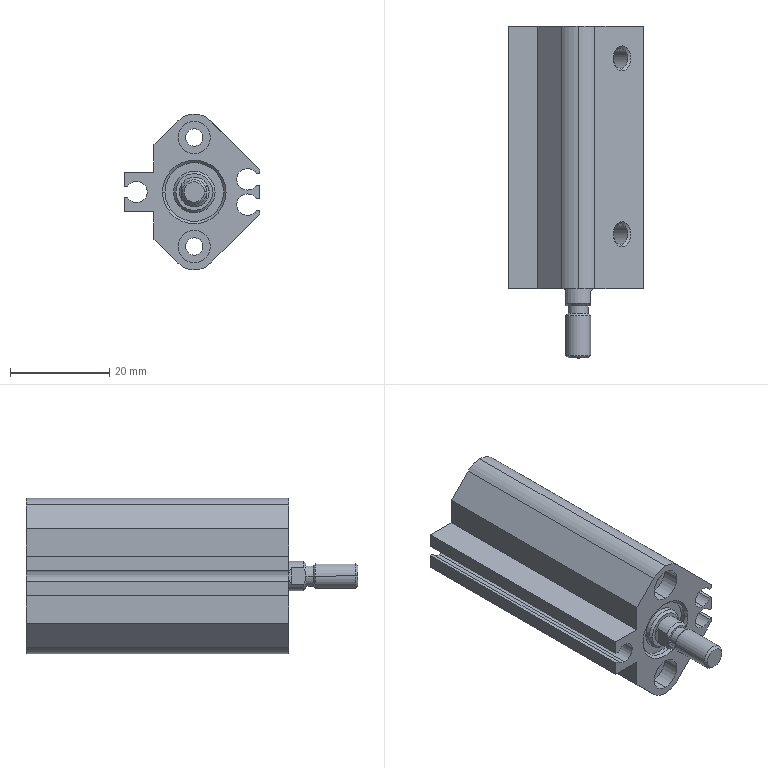Component | SolidWorks | cylinder_cdq2b12-25dm.stp-1 | 2 solids | 106 faces | volume 25433 mm3 | cylinder 49 | plane 39 | cone 18 | commonest cylinder face diameters 4.3 x9 6.5 x8 5 x6 9.446 x4 11.84 x4 8.4 x4 3.5 x4 4.132 x4